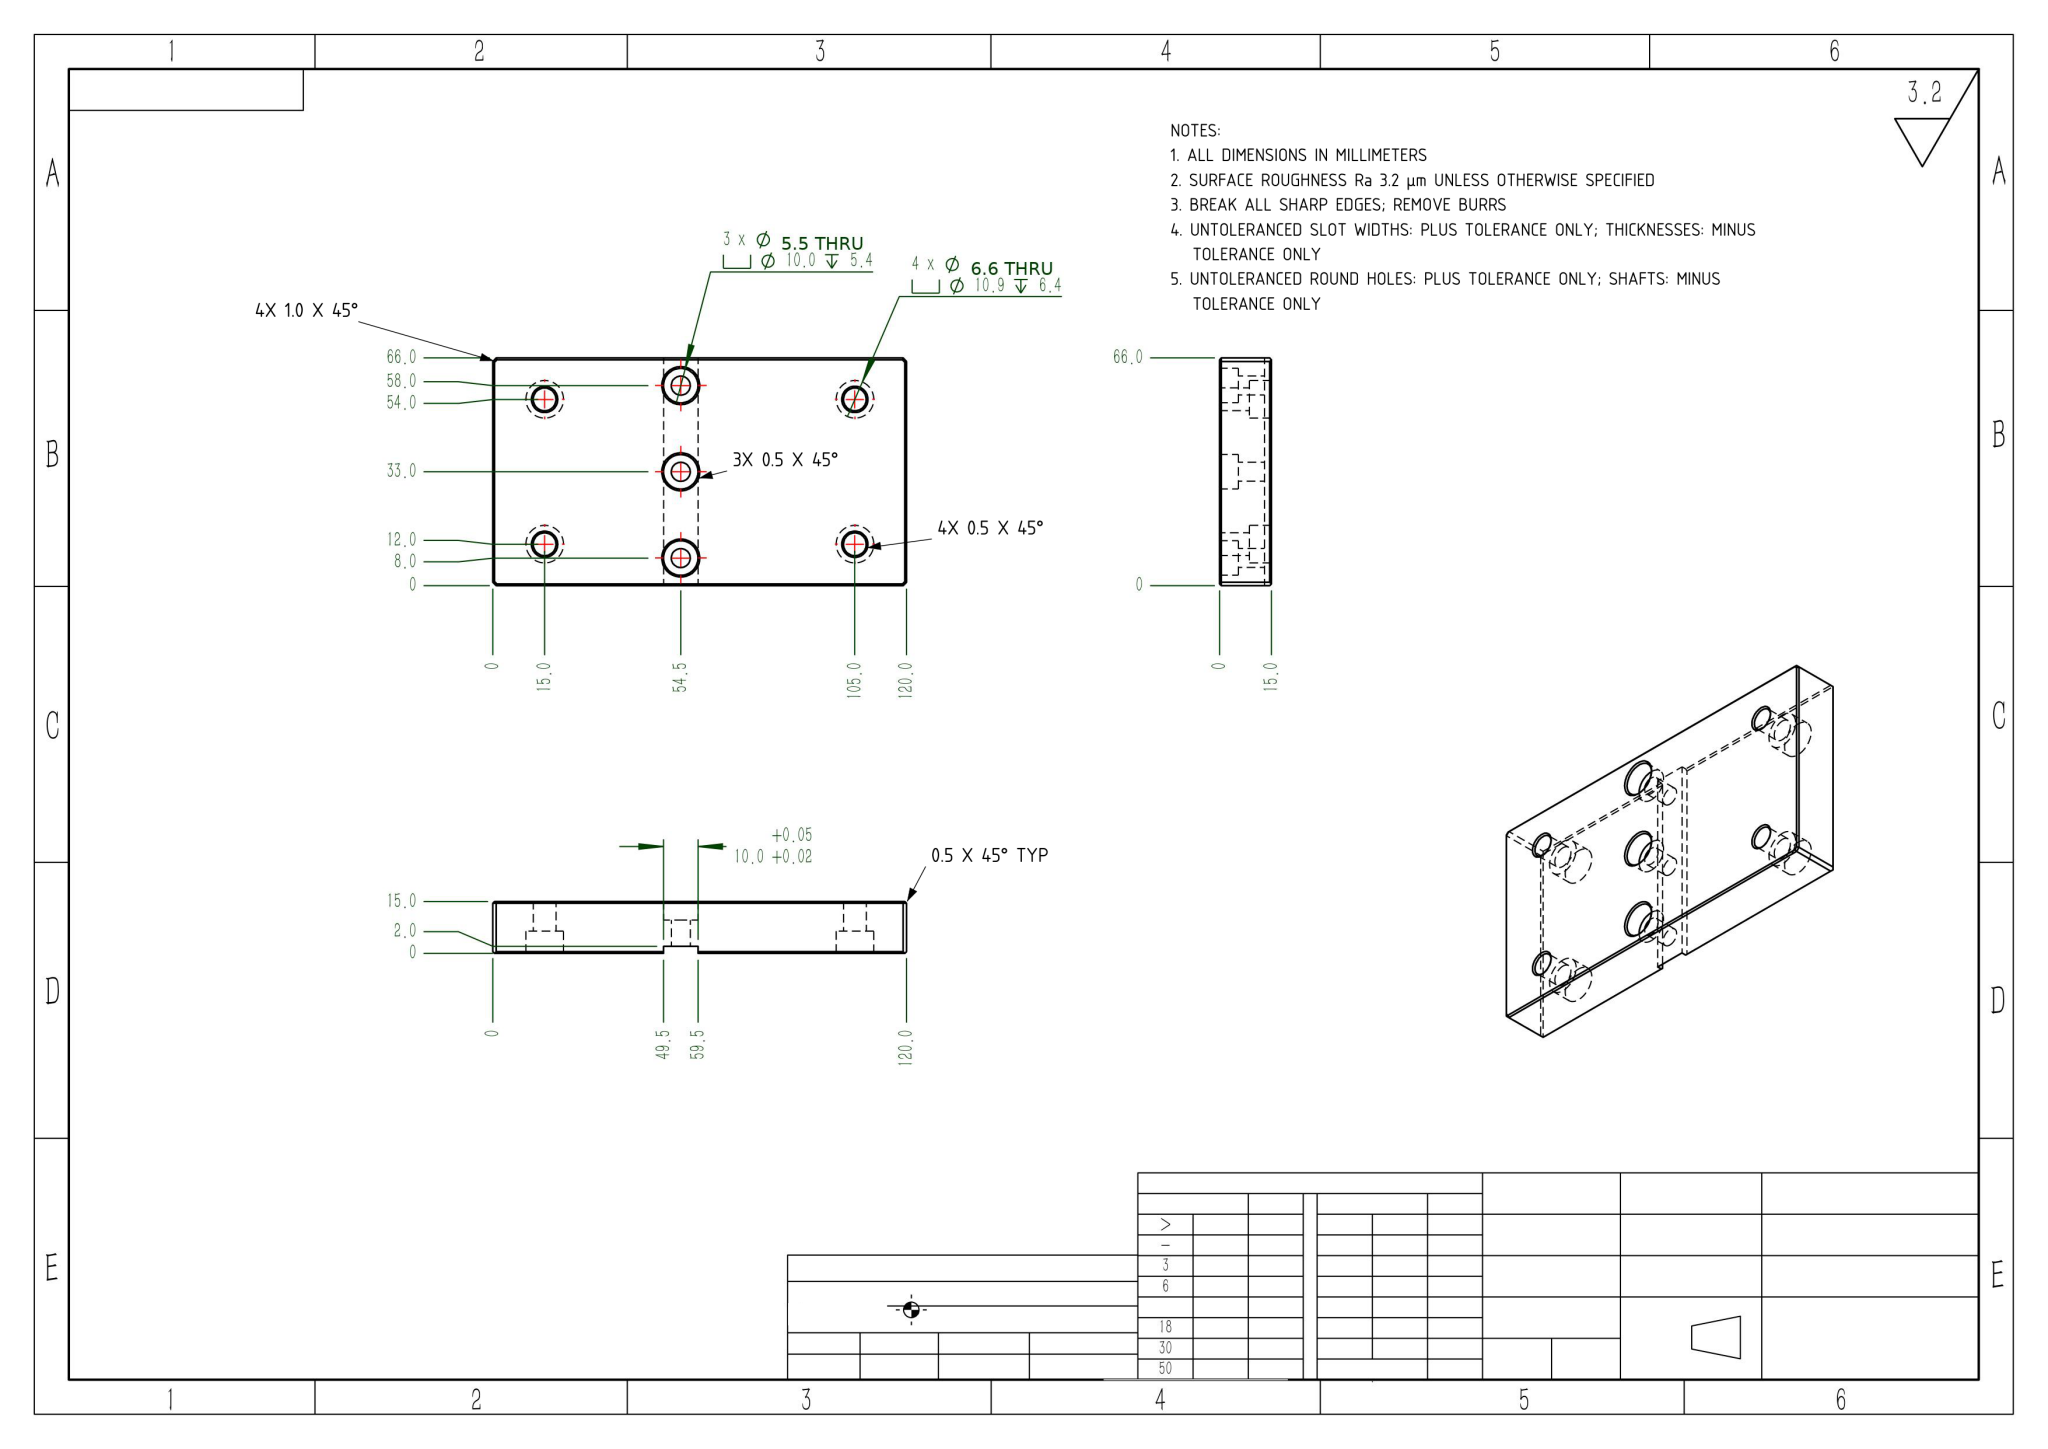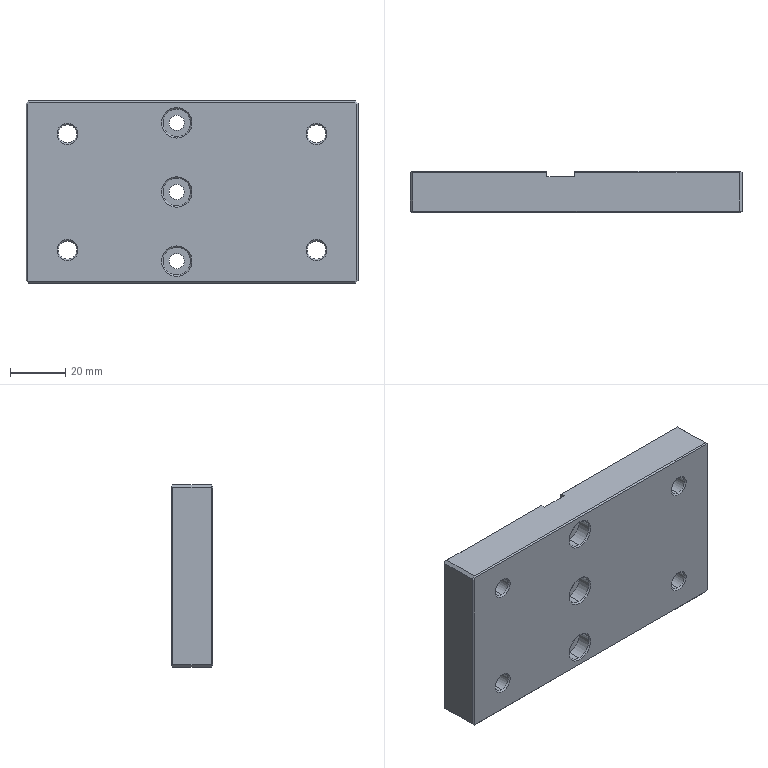Part | NX | mm | Right-Angle Seven-Hole Bracket | 1 solid | 77 faces | box 120 x 15 x 66 mm | volume 111958 mm3 | plane 35 | cylinder 28 | cone 14 | commonest cylinder face diameters 10.9 x8 6.6 x8 10 x6 5.5 x6